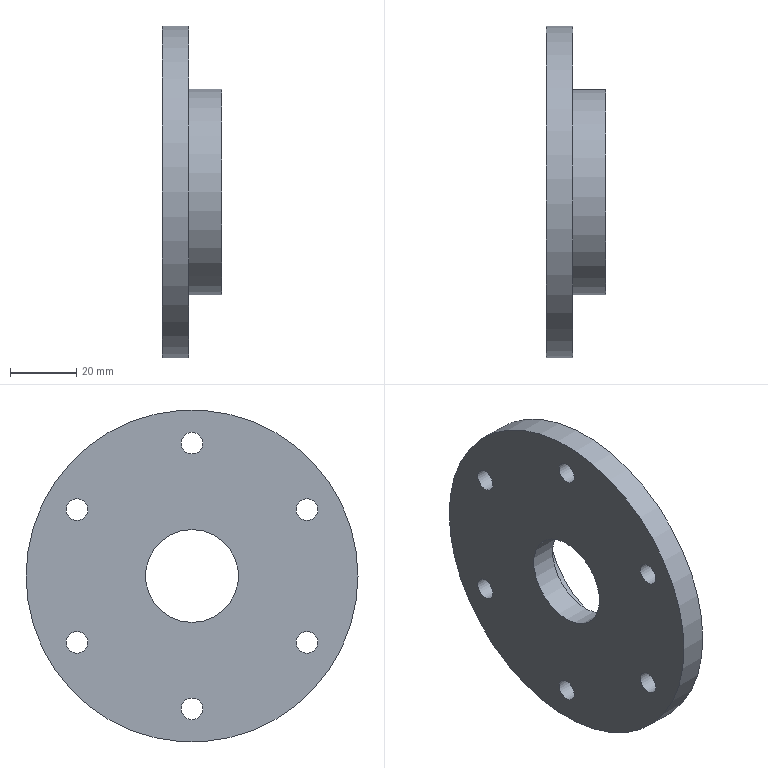Component | NX | DADUANTOUGAI | 1 solid | 14 faces | volume 66674 mm3 | cylinder 9 | plane 4 | cone 1 | commonest cylinder face diameters 6.5 x6 100 x1 62 x1 28 x1